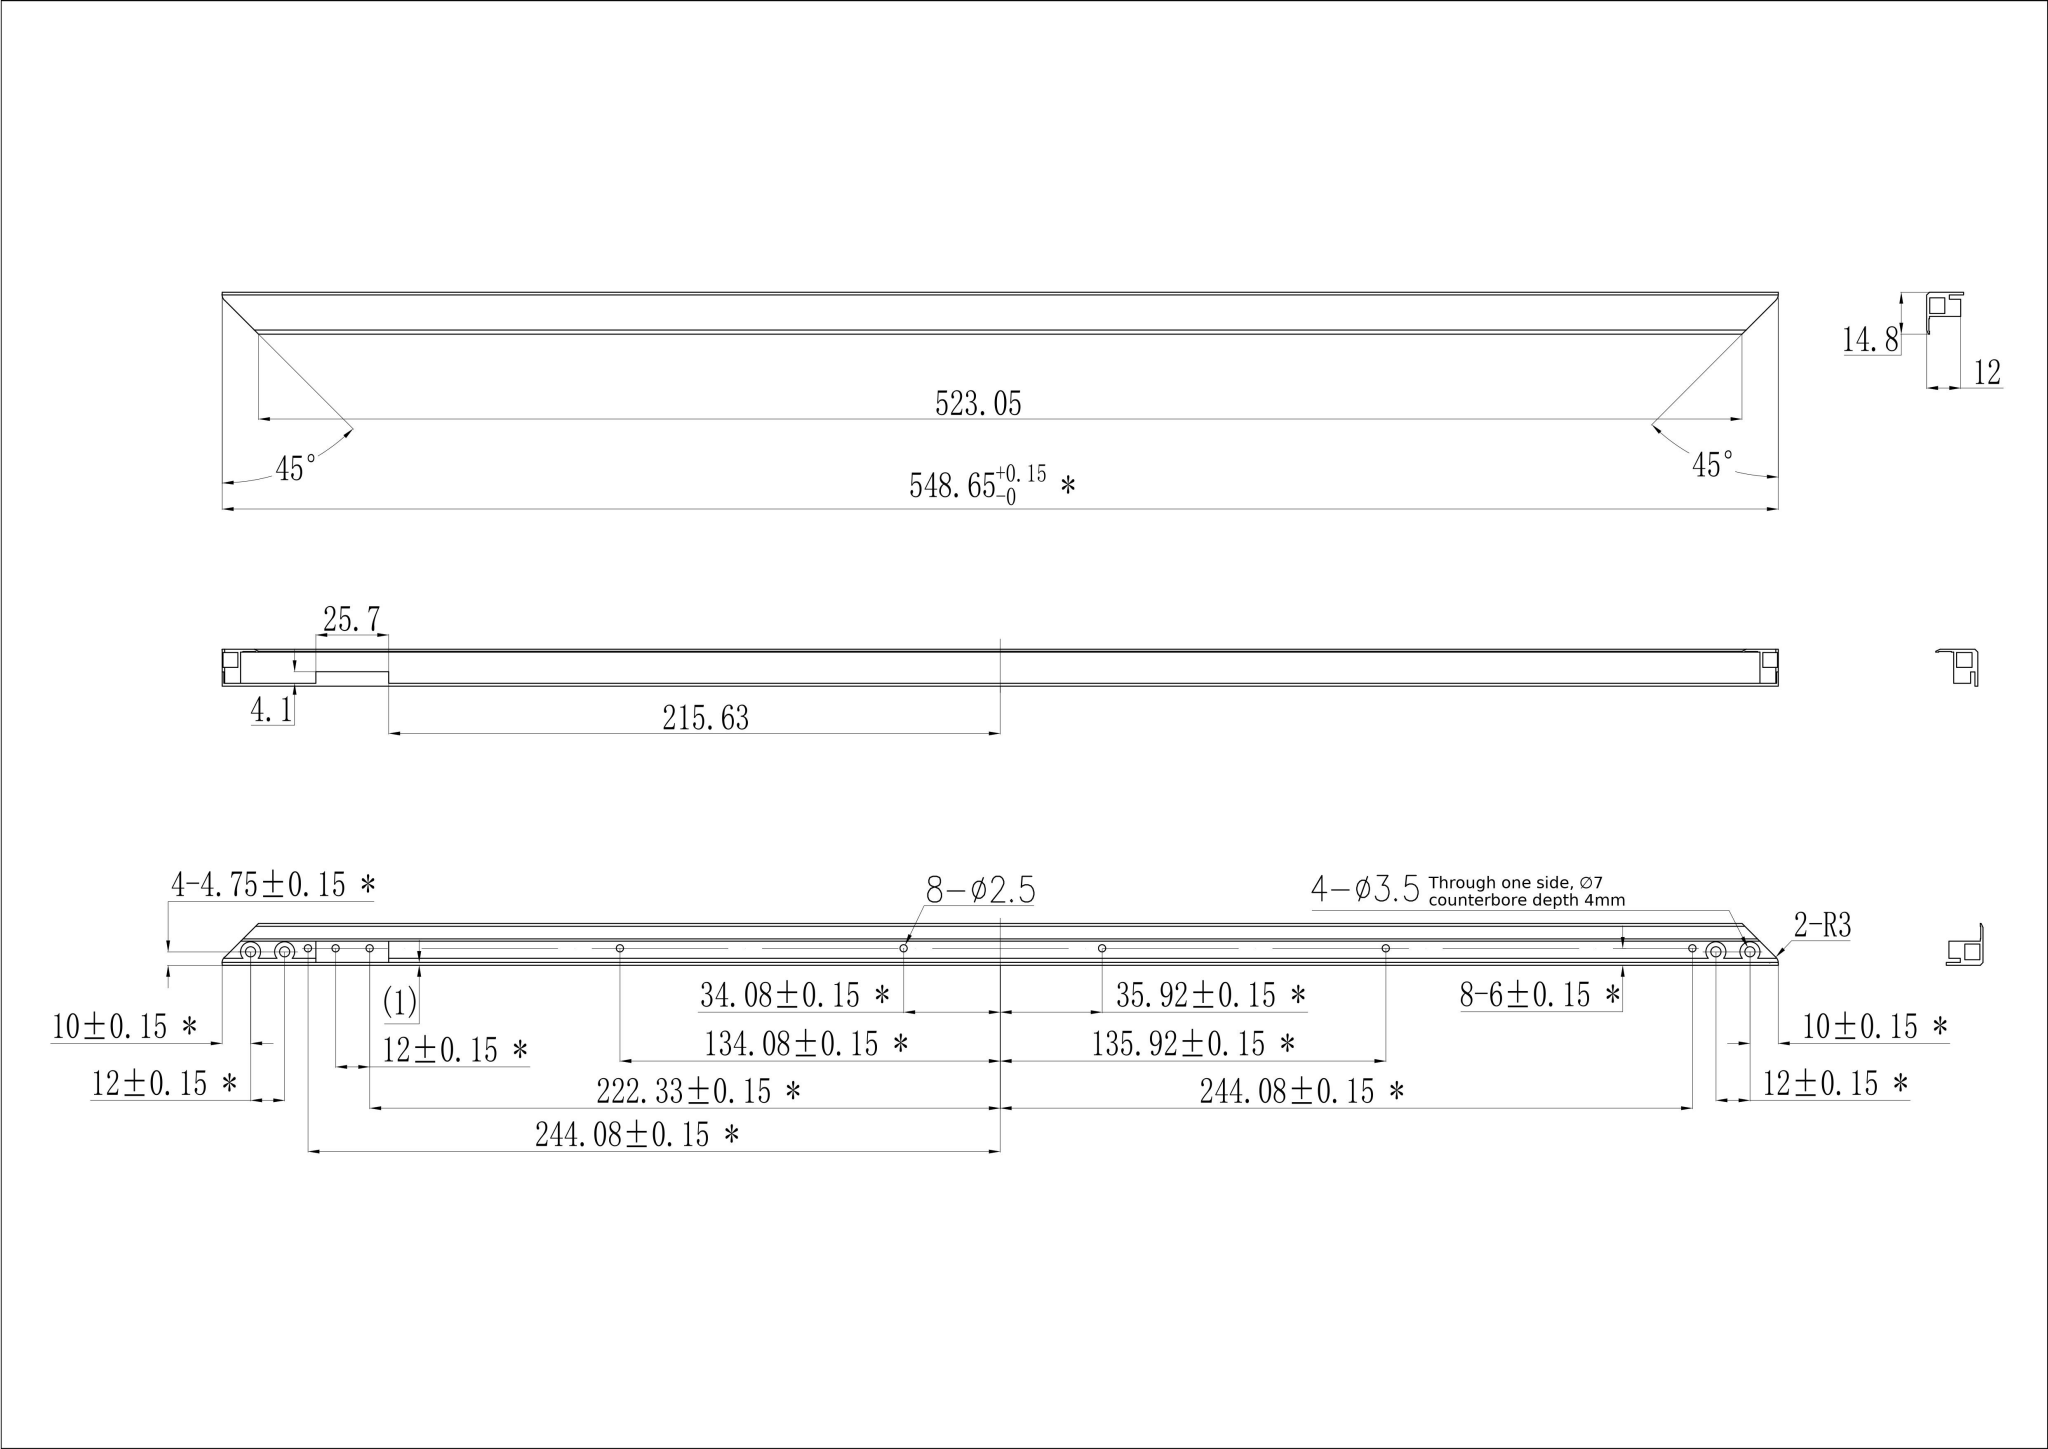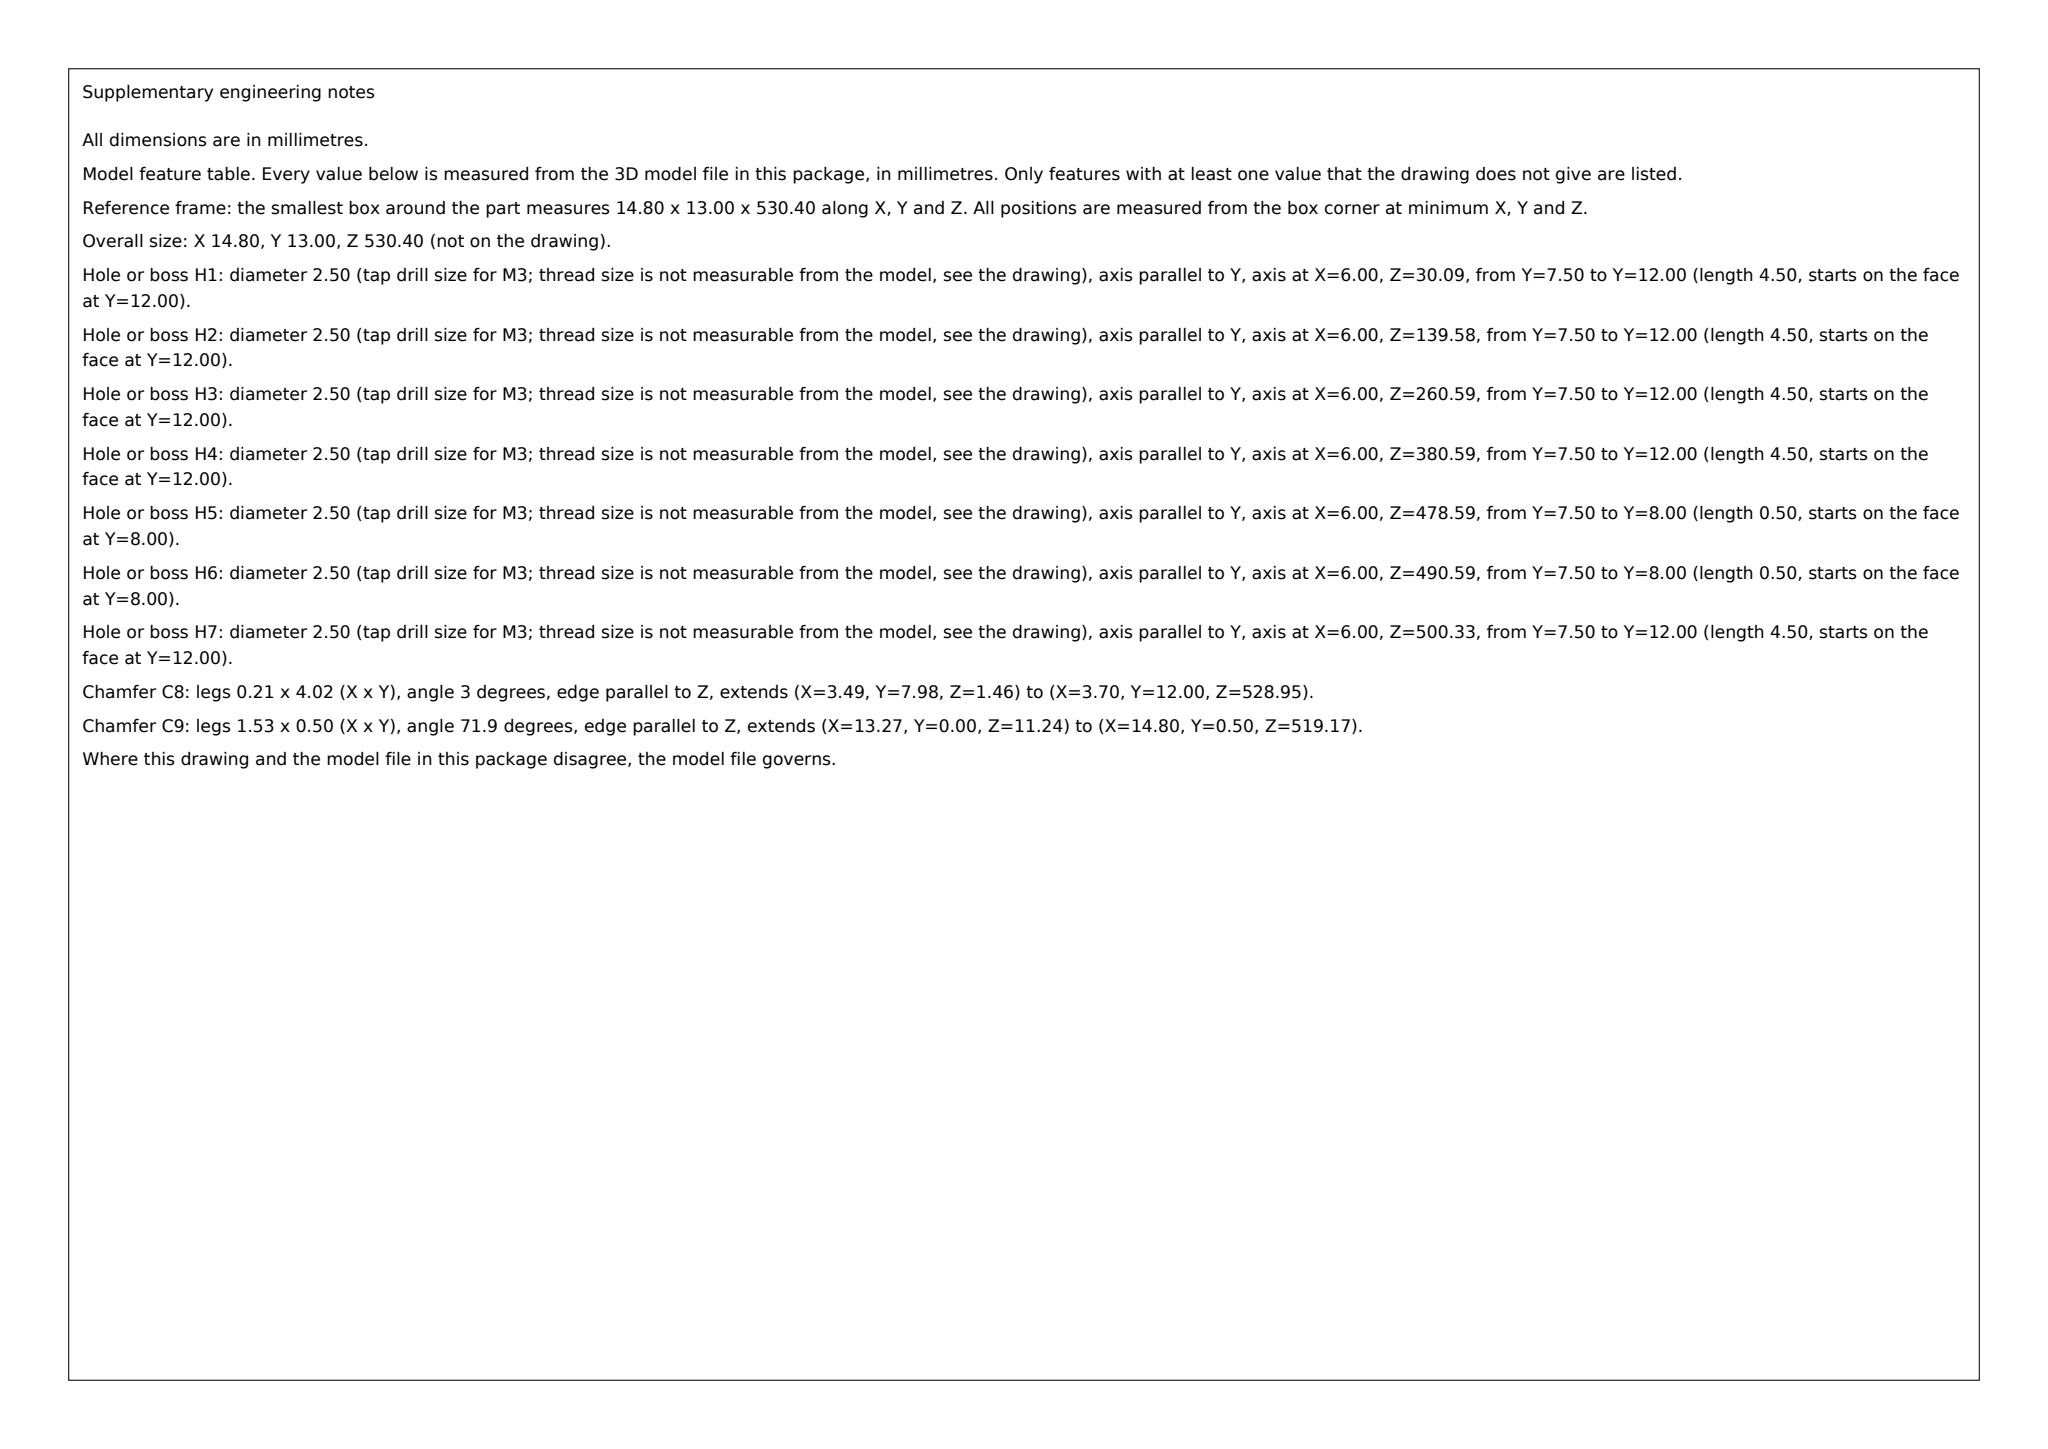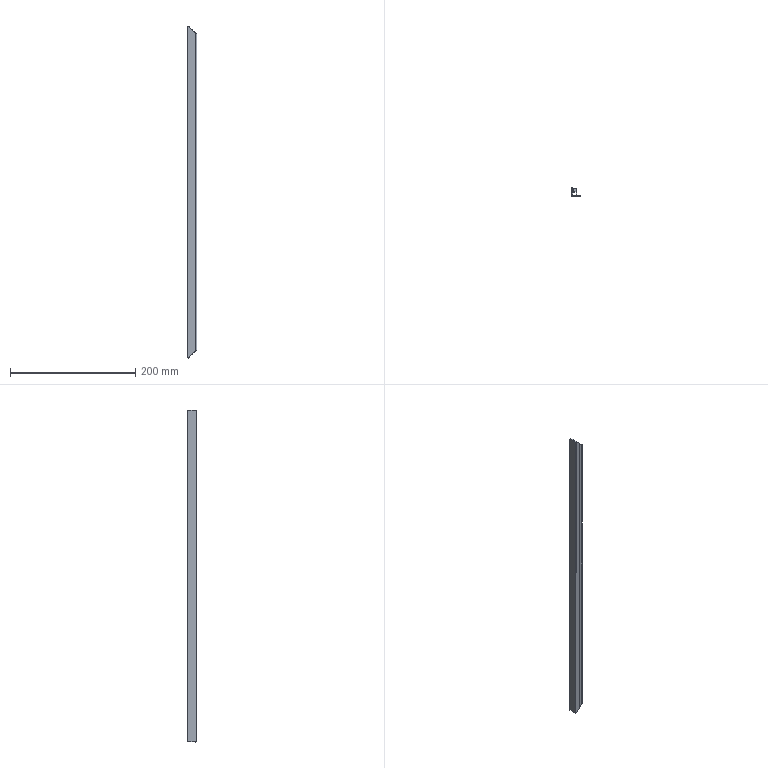Part | SolidWorks | mm | 1 solid | 44 faces | box 14.8 x 13 x 530.4 mm | volume 38168 mm3 | plane 30 | cylinder 14 | commonest cylinder face diameters 2.5 x14